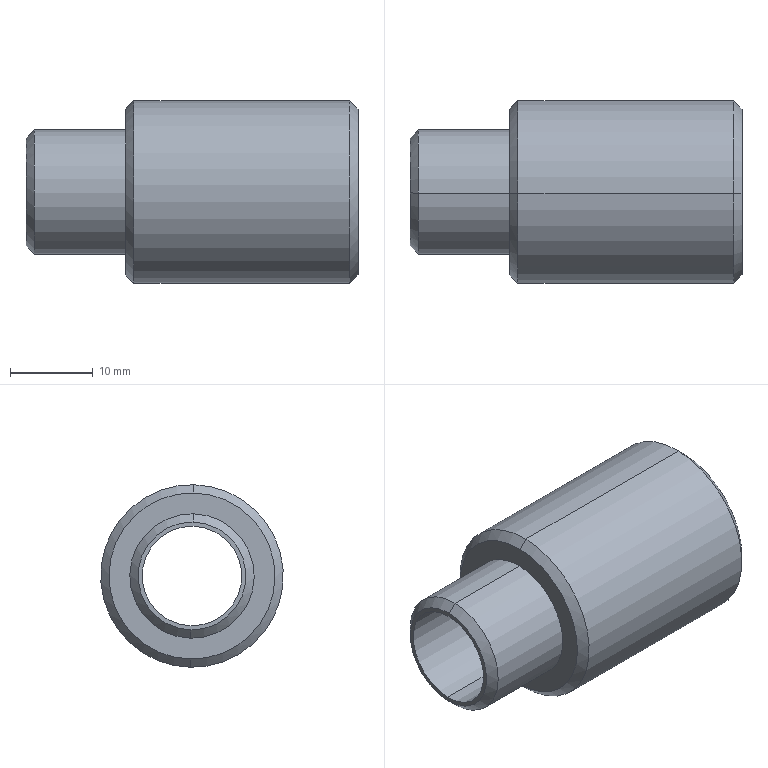Component | SolidWorks | HighVoltageCabinetFrameAssembly-1_FrameFixingSleeve-1 | 1 solid | 18 faces | box 40 x 22 x 22 mm | volume 4758 mm3 | cylinder 8 | cone 6 | plane 4 | commonest cylinder face diameters 18 x2 12 x2 15 x2 22 x2
build123d program:
from build123d import *

# Parameters (mm, degrees)
CHAMFER1_SIZE = 1


with BuildPart() as part:
    # Sketch1 → Revolve1 (revolve)
    with BuildSketch(Plane.XY, mode=Mode.PRIVATE) as revolve1_sk:
        Polygon((0, 11), (28, 11), (28, 7.5), (40, 7.5), (40, 6), (24, 6), (24, 9), (0, 9), align=None)
    revolve(revolve1_sk.sketch.rotate(Axis((0, 0, 0), (1, 0, 0)), 90), axis=Axis((0, 0, 0), (1, 0, 0)))

    # Chamfer1
    chamfer1_edges = [part.edges().sort_by_distance(p)[0] for p in [
        (40, 0, -7.5),
        (28, 0, -11),
        (0, 0, -11),
    ]]
    chamfer(chamfer1_edges, length=CHAMFER1_SIZE)


solid = part.part

# Placed as in the assembly
solid = solid.moved(Location((-1255.437, 161.417, 915.27), (-180, 0, 180)))
STEP:
#1=CARTESIAN_POINT('',(-49.427,6.347,36.428));
#2=VERTEX_POINT('',#1);
#3=CARTESIAN_POINT('',(-49.427,6.363,35.641));
#4=VERTEX_POINT('',#3);
#5=CARTESIAN_POINT('',(-49.427,6.355,36.034));
#6=DIRECTION('',(1.,0.,-0.));
#7=DIRECTION('',(0.,0.01928,-0.9998));
#8=AXIS2_PLACEMENT_3D('',#5,#6,#7);
#9=CIRCLE('',#8,0.3937);
#10=EDGE_CURVE('',#2,#4,#9,.T.);
#11=ORIENTED_EDGE('',*,*,#10,.F.);
#12=CARTESIAN_POINT('',(-49.466,6.347,36.467));
#13=VERTEX_POINT('',#12);
#14=CARTESIAN_POINT('',(-49.427,6.347,36.428));
#15=DIRECTION('',(-0.7071,-0.01364,0.707));
#16=VECTOR('',#15,39.37);
#17=LINE('',#14,#16);
#18=EDGE_CURVE('',#2,#13,#17,.T.);
#19=ORIENTED_EDGE('',*,*,#18,.T.);
#20=CARTESIAN_POINT('',(-49.466,6.363,35.601));
#21=VERTEX_POINT('',#20);
#22=CARTESIAN_POINT('',(-49.466,6.355,36.034));
#23=DIRECTION('',(-1.,-0.,0.));
#24=DIRECTION('',(0.,0.01928,-0.9998));
#25=AXIS2_PLACEMENT_3D('',#22,#23,#24);
#26=CIRCLE('',#25,0.4331);
#27=EDGE_CURVE('',#21,#13,#26,.T.);
#28=ORIENTED_EDGE('',*,*,#27,.F.);
#29=CARTESIAN_POINT('',(-49.427,6.363,35.641));
#30=DIRECTION('',(-0.7071,0.01364,-0.707));
#31=VECTOR('',#30,39.37);
#32=LINE('',#29,#31);
#33=EDGE_CURVE('',#4,#21,#32,.T.);
#34=ORIENTED_EDGE('',*,*,#33,.F.);
#35=EDGE_LOOP('',(#11,#19,#28,#34));
#36=FACE_OUTER_BOUND('',#35,.T.);
#37=CARTESIAN_POINT('',(-49.427,6.355,36.034));
#38=DIRECTION('',(-1.,-0.,0.));
#39=DIRECTION('',(0.,0.01928,-0.9998));
#40=AXIS2_PLACEMENT_3D('',#37,#38,#39);
#41=CONICAL_SURFACE('',#40,0.3937,0.7854);
#42=ADVANCED_FACE('',(#36),#41,.T.);
#43=CARTESIAN_POINT('',(-50.529,6.363,35.641));
#44=VERTEX_POINT('',#43);
#45=CARTESIAN_POINT('',(-50.529,6.347,36.428));
#46=VERTEX_POINT('',#45);
#47=CARTESIAN_POINT('',(-50.529,6.355,36.034));
#48=DIRECTION('',(-1.,-0.,0.));
#49=DIRECTION('',(0.,-0.01928,0.9998));
#50=AXIS2_PLACEMENT_3D('',#47,#48,#49);
#51=CIRCLE('',#50,0.3937);
#52=EDGE_CURVE('',#44,#46,#51,.T.);
#53=ORIENTED_EDGE('',*,*,#52,.F.);
#54=CARTESIAN_POINT('',(-50.49,6.363,35.601));
#55=VERTEX_POINT('',#54);
#56=CARTESIAN_POINT('',(-50.49,6.363,35.601));
#57=DIRECTION('',(0.7071,0.01364,-0.707));
#58=VECTOR('',#57,39.37);
#59=LINE('',#56,#58);
#60=EDGE_CURVE('',#44,#55,#59,.T.);
#61=ORIENTED_EDGE('',*,*,#60,.T.);
#62=CARTESIAN_POINT('',(-50.49,6.347,36.467));
#63=VERTEX_POINT('',#62);
#64=CARTESIAN_POINT('',(-50.49,6.355,36.034));
#65=DIRECTION('',(1.,0.,-0.));
#66=DIRECTION('',(0.,-0.01928,0.9998));
#67=AXIS2_PLACEMENT_3D('',#64,#65,#66);
#68=CIRCLE('',#67,0.4331);
#69=EDGE_CURVE('',#63,#55,#68,.T.);
#70=ORIENTED_EDGE('',*,*,#69,.F.);
#71=CARTESIAN_POINT('',(-50.49,6.347,36.467));
#72=DIRECTION('',(0.7071,-0.01364,0.707));
#73=VECTOR('',#72,39.37);
#74=LINE('',#71,#73);
#75=EDGE_CURVE('',#46,#63,#74,.T.);
#76=ORIENTED_EDGE('',*,*,#75,.F.);
#77=EDGE_LOOP('',(#53,#61,#70,#76));
#78=FACE_OUTER_BOUND('',#77,.T.);
#79=CARTESIAN_POINT('',(-50.49,6.355,36.034));
#80=DIRECTION('',(1.,0.,-0.));
#81=DIRECTION('',(0.,-0.01928,0.9998));
#82=AXIS2_PLACEMENT_3D('',#79,#80,#81);
#83=CONICAL_SURFACE('',#82,0.4331,0.7854);
#84=ADVANCED_FACE('',(#78),#83,.T.);
#85=CARTESIAN_POINT('',(-51.001,6.36,35.778));
#86=VERTEX_POINT('',#85);
#87=CARTESIAN_POINT('',(-51.001,6.35,36.29));
#88=VERTEX_POINT('',#87);
#89=CARTESIAN_POINT('',(-51.001,6.355,36.034));
#90=DIRECTION('',(-1.,-0.,0.));
#91=DIRECTION('',(0.,-0.01928,0.9998));
#92=AXIS2_PLACEMENT_3D('',#89,#90,#91);
#93=CIRCLE('',#92,0.2559);
#94=EDGE_CURVE('',#86,#88,#93,.T.);
#95=ORIENTED_EDGE('',*,*,#94,.F.);
#96=CARTESIAN_POINT('',(-50.962,6.361,35.739));
#97=VERTEX_POINT('',#96);
#98=CARTESIAN_POINT('',(-50.962,6.361,35.739));
#99=DIRECTION('',(0.7071,0.01364,-0.707));
#100=VECTOR('',#99,39.37);
#101=LINE('',#98,#100);
#102=EDGE_CURVE('',#86,#97,#101,.T.);
#103=ORIENTED_EDGE('',*,*,#102,.T.);
#104=CARTESIAN_POINT('',(-50.962,6.349,36.329));
#105=VERTEX_POINT('',#104);
#106=CARTESIAN_POINT('',(-50.962,6.355,36.034));
#107=DIRECTION('',(1.,0.,-0.));
#108=DIRECTION('',(0.,-0.01928,0.9998));
#109=AXIS2_PLACEMENT_3D('',#106,#107,#108);
#110=CIRCLE('',#109,0.2953);
#111=EDGE_CURVE('',#105,#97,#110,.T.);
#112=ORIENTED_EDGE('',*,*,#111,.F.);
#113=CARTESIAN_POINT('',(-50.962,6.349,36.329));
#114=DIRECTION('',(0.7071,-0.01364,0.707));
#115=VECTOR('',#114,39.37);
#116=LINE('',#113,#115);
#117=EDGE_CURVE('',#88,#105,#116,.T.);
#118=ORIENTED_EDGE('',*,*,#117,.F.);
#119=EDGE_LOOP('',(#95,#103,#112,#118));
#120=FACE_OUTER_BOUND('',#119,.T.);
#121=CARTESIAN_POINT('',(-50.962,6.355,36.034));
#122=DIRECTION('',(1.,0.,-0.));
#123=DIRECTION('',(0.,-0.01928,0.9998));
#124=AXIS2_PLACEMENT_3D('',#121,#122,#123);
#125=CONICAL_SURFACE('',#124,0.2953,0.7854);
#126=ADVANCED_FACE('',(#120),#125,.T.);
#127=CARTESIAN_POINT('',(-50.372,6.362,35.68));
#128=VERTEX_POINT('',#127);
#129=CARTESIAN_POINT('',(-50.372,6.348,36.389));
#130=VERTEX_POINT('',#129);
#131=CARTESIAN_POINT('',(-50.372,6.355,36.034));
#132=DIRECTION('',(1.,0.,-0.));
#133=DIRECTION('',(0.,-0.01928,0.9998));
#134=AXIS2_PLACEMENT_3D('',#131,#132,#133);
#135=CIRCLE('',#134,0.3543);
#136=EDGE_CURVE('',#128,#130,#135,.T.);
#137=ORIENTED_EDGE('',*,*,#136,.F.);
#138=CARTESIAN_POINT('',(-49.427,6.362,35.68));
#139=VERTEX_POINT('',#138);
#140=CARTESIAN_POINT('',(-49.427,6.362,35.68));
#141=DIRECTION('',(1.,0.,-0.));
#142=VECTOR('',#141,39.37);
#143=LINE('',#140,#142);
#144=EDGE_CURVE('',#128,#139,#143,.T.);
#145=ORIENTED_EDGE('',*,*,#144,.T.);
#146=CARTESIAN_POINT('',(-49.427,6.348,36.389));
#147=VERTEX_POINT('',#146);
#148=CARTESIAN_POINT('',(-49.427,6.355,36.034));
#149=DIRECTION('',(1.,0.,-0.));
#150=DIRECTION('',(0.,-0.01928,0.9998));
#151=AXIS2_PLACEMENT_3D('',#148,#149,#150);
#152=CIRCLE('',#151,0.3543);
#153=EDGE_CURVE('',#139,#147,#152,.T.);
#154=ORIENTED_EDGE('',*,*,#153,.T.);
#155=CARTESIAN_POINT('',(-49.427,6.348,36.389));
#156=DIRECTION('',(1.,0.,-0.));
#157=VECTOR('',#156,39.37);
#158=LINE('',#155,#157);
#159=EDGE_CURVE('',#130,#147,#158,.T.);
#160=ORIENTED_EDGE('',*,*,#159,.F.);
#161=EDGE_LOOP('',(#137,#145,#154,#160));
#162=FACE_OUTER_BOUND('',#161,.T.);
#163=CARTESIAN_POINT('',(-49.427,6.355,36.034));
#164=DIRECTION('',(1.,0.,-0.));
#165=DIRECTION('',(0.,-0.01928,0.9998));
#166=AXIS2_PLACEMENT_3D('',#163,#164,#165);
#167=CYLINDRICAL_SURFACE('',#166,0.3543);
#168=ADVANCED_FACE('',(#162),#167,.F.);
#169=CARTESIAN_POINT('',(-51.001,6.36,35.798));
#170=VERTEX_POINT('',#169);
#171=CARTESIAN_POINT('',(-51.001,6.35,36.27));
#172=VERTEX_POINT('',#171);
#173=CARTESIAN_POINT('',(-51.001,6.355,36.034));
#174=DIRECTION('',(1.,0.,-0.));
#175=DIRECTION('',(0.,-0.01928,0.9998));
#176=AXIS2_PLACEMENT_3D('',#173,#174,#175);
#177=CIRCLE('',#176,0.2362);
#178=EDGE_CURVE('',#170,#172,#177,.T.);
#179=ORIENTED_EDGE('',*,*,#178,.F.);
#180=CARTESIAN_POINT('',(-50.372,6.36,35.798));
#181=VERTEX_POINT('',#180);
#182=CARTESIAN_POINT('',(-49.427,6.36,35.798));
#183=DIRECTION('',(1.,0.,-0.));
#184=VECTOR('',#183,39.37);
#185=LINE('',#182,#184);
#186=EDGE_CURVE('',#170,#181,#185,.T.);
#187=ORIENTED_EDGE('',*,*,#186,.T.);
#188=CARTESIAN_POINT('',(-50.372,6.35,36.27));
#189=VERTEX_POINT('',#188);
#190=CARTESIAN_POINT('',(-50.372,6.355,36.034));
#191=DIRECTION('',(1.,0.,-0.));
#192=DIRECTION('',(0.,-0.01928,0.9998));
#193=AXIS2_PLACEMENT_3D('',#190,#191,#192);
#194=CIRCLE('',#193,0.2362);
#195=EDGE_CURVE('',#181,#189,#194,.T.);
#196=ORIENTED_EDGE('',*,*,#195,.T.);
#197=CARTESIAN_POINT('',(-49.427,6.35,36.27));
#198=DIRECTION('',(1.,0.,-0.));
#199=VECTOR('',#198,39.37);
#200=LINE('',#197,#199);
#201=EDGE_CURVE('',#172,#189,#200,.T.);
#202=ORIENTED_EDGE('',*,*,#201,.F.);
#203=EDGE_LOOP('',(#179,#187,#196,#202));
#204=FACE_OUTER_BOUND('',#203,.T.);
#205=CARTESIAN_POINT('',(-49.427,6.355,36.034));
#206=DIRECTION('',(1.,0.,-0.));
#207=DIRECTION('',(0.,-0.01928,0.9998));
#208=AXIS2_PLACEMENT_3D('',#205,#206,#207);
#209=CYLINDRICAL_SURFACE('',#208,0.2362);
#210=ADVANCED_FACE('',(#204),#209,.F.);
#211=ORIENTED_EDGE('',*,*,#111,.T.);
#212=CARTESIAN_POINT('',(-50.529,6.361,35.739));
#213=VERTEX_POINT('',#212);
#214=CARTESIAN_POINT('',(-49.427,6.361,35.739));
#215=DIRECTION('',(1.,0.,-0.));
#216=VECTOR('',#215,39.37);
#217=LINE('',#214,#216);
#218=EDGE_CURVE('',#97,#213,#217,.T.);
#219=ORIENTED_EDGE('',*,*,#218,.T.);
#220=CARTESIAN_POINT('',(-50.529,6.349,36.329));
#221=VERTEX_POINT('',#220);
#222=CARTESIAN_POINT('',(-50.529,6.355,36.034));
#223=DIRECTION('',(1.,0.,-0.));
#224=DIRECTION('',(0.,-0.01928,0.9998));
#225=AXIS2_PLACEMENT_3D('',#222,#223,#224);
#226=CIRCLE('',#225,0.2953);
#227=EDGE_CURVE('',#221,#213,#226,.T.);
#228=ORIENTED_EDGE('',*,*,#227,.F.);
#229=CARTESIAN_POINT('',(-49.427,6.349,36.329));
#230=DIRECTION('',(1.,0.,-0.));
#231=VECTOR('',#230,39.37);
#232=LINE('',#229,#231);
#233=EDGE_CURVE('',#105,#221,#232,.T.);
#234=ORIENTED_EDGE('',*,*,#233,.F.);
#235=EDGE_LOOP('',(#211,#219,#228,#234));
#236=FACE_OUTER_BOUND('',#235,.T.);
#237=CARTESIAN_POINT('',(-49.427,6.355,36.034));
#238=DIRECTION('',(1.,0.,-0.));
#239=DIRECTION('',(0.,-0.01928,0.9998));
#240=AXIS2_PLACEMENT_3D('',#237,#238,#239);
#241=CYLINDRICAL_SURFACE('',#240,0.2953);
#242=ADVANCED_FACE('',(#236),#241,.T.);
#243=ORIENTED_EDGE('',*,*,#69,.T.);
#244=CARTESIAN_POINT('',(-49.427,6.363,35.601));
#245=DIRECTION('',(1.,0.,-0.));
#246=VECTOR('',#245,39.37);
#247=LINE('',#244,#246);
#248=EDGE_CURVE('',#55,#21,#247,.T.);
#249=ORIENTED_EDGE('',*,*,#248,.T.);
#250=ORIENTED_EDGE('',*,*,#27,.T.);
#251=CARTESIAN_POINT('',(-49.427,6.347,36.467));
#252=DIRECTION('',(1.,0.,-0.));
#253=VECTOR('',#252,39.37);
#254=LINE('',#251,#253);
#255=EDGE_CURVE('',#63,#13,#254,.T.);
#256=ORIENTED_EDGE('',*,*,#255,.F.);
#257=EDGE_LOOP('',(#243,#249,#250,#256));
#258=FACE_OUTER_BOUND('',#257,.T.);
#259=CARTESIAN_POINT('',(-49.427,6.355,36.034));
#260=DIRECTION('',(1.,0.,-0.));
#261=DIRECTION('',(0.,-0.01928,0.9998));
#262=AXIS2_PLACEMENT_3D('',#259,#260,#261);
#263=CYLINDRICAL_SURFACE('',#262,0.4331);
#264=ADVANCED_FACE('',(#258),#263,.T.);
#265=CARTESIAN_POINT('',(-49.427,6.355,36.034));
#266=DIRECTION('',(1.,0.,-0.));
#267=DIRECTION('',(0.,0.01928,-0.9998));
#268=AXIS2_PLACEMENT_3D('',#265,#266,#267);
#269=CIRCLE('',#268,0.3937);
#270=EDGE_CURVE('',#4,#2,#269,.T.);
#271=ORIENTED_EDGE('',*,*,#270,.T.);
#272=ORIENTED_EDGE('',*,*,#10,.T.);
#273=EDGE_LOOP('',(#271,#272));
#274=FACE_OUTER_BOUND('',#273,.T.);
#275=CARTESIAN_POINT('',(-49.427,6.355,36.034));
#276=DIRECTION('',(1.,0.,-0.));
#277=DIRECTION('',(0.,-0.01928,0.9998));
#278=AXIS2_PLACEMENT_3D('',#275,#276,#277);
#279=CIRCLE('',#278,0.3543);
#280=EDGE_CURVE('',#147,#139,#279,.T.);
#281=ORIENTED_EDGE('',*,*,#280,.F.);
#282=ORIENTED_EDGE('',*,*,#153,.F.);
#283=EDGE_LOOP('',(#281,#282));
#284=FACE_BOUND('',#283,.T.);
#285=CARTESIAN_POINT('',(-49.427,6.001,36.027));
#286=DIRECTION('',(-1.,-0.,-0.));
#287=DIRECTION('',(0.,0.01928,-0.9998));
#288=AXIS2_PLACEMENT_3D('',#285,#286,#287);
#289=PLANE('',#288);
#290=ADVANCED_FACE('',(#274,#284),#289,.F.);
#291=ORIENTED_EDGE('',*,*,#248,.F.);
#292=CARTESIAN_POINT('',(-50.49,6.355,36.034));
#293=DIRECTION('',(1.,0.,-0.));
#294=DIRECTION('',(0.,-0.01928,0.9998));
#295=AXIS2_PLACEMENT_3D('',#292,#293,#294);
#296=CIRCLE('',#295,0.4331);
#297=EDGE_CURVE('',#55,#63,#296,.T.);
#298=ORIENTED_EDGE('',*,*,#297,.T.);
#299=ORIENTED_EDGE('',*,*,#255,.T.);
#300=CARTESIAN_POINT('',(-49.466,6.355,36.034));
#301=DIRECTION('',(-1.,-0.,0.));
#302=DIRECTION('',(0.,0.01928,-0.9998));
#303=AXIS2_PLACEMENT_3D('',#300,#301,#302);
#304=CIRCLE('',#303,0.4331);
#305=EDGE_CURVE('',#13,#21,#304,.T.);
#306=ORIENTED_EDGE('',*,*,#305,.T.);
#307=EDGE_LOOP('',(#291,#298,#299,#306));
#308=FACE_OUTER_BOUND('',#307,.T.);
#309=CARTESIAN_POINT('',(-49.427,6.355,36.034));
#310=DIRECTION('',(1.,0.,-0.));
#311=DIRECTION('',(0.,-0.01928,0.9998));
#312=AXIS2_PLACEMENT_3D('',#309,#310,#311);
#313=CYLINDRICAL_SURFACE('',#312,0.4331);
#314=ADVANCED_FACE('',(#308),#313,.T.);
#315=CARTESIAN_POINT('',(-50.529,6.355,36.034));
#316=DIRECTION('',(-1.,-0.,0.));
#317=DIRECTION('',(0.,-0.01928,0.9998));
#318=AXIS2_PLACEMENT_3D('',#315,#316,#317);
#319=CIRCLE('',#318,0.3937);
#320=EDGE_CURVE('',#46,#44,#319,.T.);
#321=ORIENTED_EDGE('',*,*,#320,.T.);
#322=ORIENTED_EDGE('',*,*,#52,.T.);
#323=EDGE_LOOP('',(#321,#322));
#324=FACE_OUTER_BOUND('',#323,.T.);
#325=ORIENTED_EDGE('',*,*,#227,.T.);
#326=CARTESIAN_POINT('',(-50.529,6.355,36.034));
#327=DIRECTION('',(1.,0.,-0.));
#328=DIRECTION('',(0.,-0.01928,0.9998));
#329=AXIS2_PLACEMENT_3D('',#326,#327,#328);
#330=CIRCLE('',#329,0.2953);
#331=EDGE_CURVE('',#213,#221,#330,.T.);
#332=ORIENTED_EDGE('',*,*,#331,.T.);
#333=EDGE_LOOP('',(#325,#332));
#334=FACE_BOUND('',#333,.T.);
#335=CARTESIAN_POINT('',(-50.529,5.922,36.026));
#336=DIRECTION('',(1.,0.,0.));
#337=DIRECTION('',(-0.,-0.01928,0.9998));
#338=AXIS2_PLACEMENT_3D('',#335,#336,#337);
#339=PLANE('',#338);
#340=ADVANCED_FACE('',(#324,#334),#339,.F.);
#341=ORIENTED_EDGE('',*,*,#218,.F.);
#342=CARTESIAN_POINT('',(-50.962,6.355,36.034));
#343=DIRECTION('',(1.,0.,-0.));
#344=DIRECTION('',(0.,-0.01928,0.9998));
#345=AXIS2_PLACEMENT_3D('',#342,#343,#344);
#346=CIRCLE('',#345,0.2953);
#347=EDGE_CURVE('',#97,#105,#346,.T.);
#348=ORIENTED_EDGE('',*,*,#347,.T.);
#349=ORIENTED_EDGE('',*,*,#233,.T.);
#350=ORIENTED_EDGE('',*,*,#331,.F.);
#351=EDGE_LOOP('',(#341,#348,#349,#350));
#352=FACE_OUTER_BOUND('',#351,.T.);
#353=CARTESIAN_POINT('',(-49.427,6.355,36.034));
#354=DIRECTION('',(1.,0.,-0.));
#355=DIRECTION('',(0.,-0.01928,0.9998));
#356=AXIS2_PLACEMENT_3D('',#353,#354,#355);
#357=CYLINDRICAL_SURFACE('',#356,0.2953);
#358=ADVANCED_FACE('',(#352),#357,.T.);
#359=CARTESIAN_POINT('',(-51.001,6.355,36.034));
#360=DIRECTION('',(-1.,-0.,0.));
#361=DIRECTION('',(0.,-0.01928,0.9998));
#362=AXIS2_PLACEMENT_3D('',#359,#360,#361);
#363=CIRCLE('',#362,0.2559);
#364=EDGE_CURVE('',#88,#86,#363,.T.);
#365=ORIENTED_EDGE('',*,*,#364,.T.);
#366=ORIENTED_EDGE('',*,*,#94,.T.);
#367=EDGE_LOOP('',(#365,#366));
#368=FACE_OUTER_BOUND('',#367,.T.);
#369=CARTESIAN_POINT('',(-51.001,6.355,36.034));
#370=DIRECTION('',(1.,0.,-0.));
#371=DIRECTION('',(0.,-0.01928,0.9998));
#372=AXIS2_PLACEMENT_3D('',#369,#370,#371);
#373=CIRCLE('',#372,0.2362);
#374=EDGE_CURVE('',#172,#170,#373,.T.);
#375=ORIENTED_EDGE('',*,*,#374,.T.);
#376=ORIENTED_EDGE('',*,*,#178,.T.);
#377=EDGE_LOOP('',(#375,#376));
#378=FACE_BOUND('',#377,.T.);
#379=CARTESIAN_POINT('',(-51.001,6.06,36.029));
#380=DIRECTION('',(1.,0.,0.));
#381=DIRECTION('',(-0.,-0.01928,0.9998));
#382=AXIS2_PLACEMENT_3D('',#379,#380,#381);
#383=PLANE('',#382);
#384=ADVANCED_FACE('',(#368,#378),#383,.F.);
#385=ORIENTED_EDGE('',*,*,#186,.F.);
#386=ORIENTED_EDGE('',*,*,#374,.F.);
#387=ORIENTED_EDGE('',*,*,#201,.T.);
#388=CARTESIAN_POINT('',(-50.372,6.355,36.034));
#389=DIRECTION('',(1.,0.,-0.));
#390=DIRECTION('',(0.,-0.01928,0.9998));
#391=AXIS2_PLACEMENT_3D('',#388,#389,#390);
#392=CIRCLE('',#391,0.2362);
#393=EDGE_CURVE('',#189,#181,#392,.T.);
#394=ORIENTED_EDGE('',*,*,#393,.T.);
#395=EDGE_LOOP('',(#385,#386,#387,#394));
#396=FACE_OUTER_BOUND('',#395,.T.);
#397=CARTESIAN_POINT('',(-49.427,6.355,36.034));
#398=DIRECTION('',(1.,0.,-0.));
#399=DIRECTION('',(0.,-0.01928,0.9998));
#400=AXIS2_PLACEMENT_3D('',#397,#398,#399);
#401=CYLINDRICAL_SURFACE('',#400,0.2362);
#402=ADVANCED_FACE('',(#396),#401,.F.);
#403=ORIENTED_EDGE('',*,*,#393,.F.);
#404=ORIENTED_EDGE('',*,*,#195,.F.);
#405=EDGE_LOOP('',(#403,#404));
#406=FACE_BOUND('',#405,.T.);
#407=CARTESIAN_POINT('',(-50.372,6.355,36.034));
#408=DIRECTION('',(1.,0.,-0.));
#409=DIRECTION('',(0.,-0.01928,0.9998));
#410=AXIS2_PLACEMENT_3D('',#407,#408,#409);
#411=CIRCLE('',#410,0.3543);
#412=EDGE_CURVE('',#130,#128,#411,.T.);
#413=ORIENTED_EDGE('',*,*,#412,.T.);
#414=ORIENTED_EDGE('',*,*,#136,.T.);
#415=EDGE_LOOP('',(#413,#414));
#416=FACE_OUTER_BOUND('',#415,.T.);
#417=CARTESIAN_POINT('',(-50.372,6.119,36.03));
#418=DIRECTION('',(-1.,-0.,-0.));
#419=DIRECTION('',(0.,0.01928,-0.9998));
#420=AXIS2_PLACEMENT_3D('',#417,#418,#419);
#421=PLANE('',#420);
#422=ADVANCED_FACE('',(#406,#416),#421,.F.);
#423=ORIENTED_EDGE('',*,*,#144,.F.);
#424=ORIENTED_EDGE('',*,*,#412,.F.);
#425=ORIENTED_EDGE('',*,*,#159,.T.);
#426=ORIENTED_EDGE('',*,*,#280,.T.);
#427=EDGE_LOOP('',(#423,#424,#425,#426));
#428=FACE_OUTER_BOUND('',#427,.T.);
#429=CARTESIAN_POINT('',(-49.427,6.355,36.034));
#430=DIRECTION('',(1.,0.,-0.));
#431=DIRECTION('',(0.,-0.01928,0.9998));
#432=AXIS2_PLACEMENT_3D('',#429,#430,#431);
#433=CYLINDRICAL_SURFACE('',#432,0.3543);
#434=ADVANCED_FACE('',(#428),#433,.F.);
#435=ORIENTED_EDGE('',*,*,#102,.F.);
#436=ORIENTED_EDGE('',*,*,#364,.F.);
#437=ORIENTED_EDGE('',*,*,#117,.T.);
#438=ORIENTED_EDGE('',*,*,#347,.F.);
#439=EDGE_LOOP('',(#435,#436,#437,#438));
#440=FACE_OUTER_BOUND('',#439,.T.);
#441=CARTESIAN_POINT('',(-50.962,6.355,36.034));
#442=DIRECTION('',(1.,0.,-0.));
#443=DIRECTION('',(0.,-0.01928,0.9998));
#444=AXIS2_PLACEMENT_3D('',#441,#442,#443);
#445=CONICAL_SURFACE('',#444,0.2953,0.7854);
#446=ADVANCED_FACE('',(#440),#445,.T.);
#447=ORIENTED_EDGE('',*,*,#60,.F.);
#448=ORIENTED_EDGE('',*,*,#320,.F.);
#449=ORIENTED_EDGE('',*,*,#75,.T.);
#450=ORIENTED_EDGE('',*,*,#297,.F.);
#451=EDGE_LOOP('',(#447,#448,#449,#450));
#452=FACE_OUTER_BOUND('',#451,.T.);
#453=CARTESIAN_POINT('',(-50.49,6.355,36.034));
#454=DIRECTION('',(1.,0.,-0.));
#455=DIRECTION('',(0.,-0.01928,0.9998));
#456=AXIS2_PLACEMENT_3D('',#453,#454,#455);
#457=CONICAL_SURFACE('',#456,0.4331,0.7854);
#458=ADVANCED_FACE('',(#452),#457,.T.);
#459=ORIENTED_EDGE('',*,*,#18,.F.);
#460=ORIENTED_EDGE('',*,*,#270,.F.);
#461=ORIENTED_EDGE('',*,*,#33,.T.);
#462=ORIENTED_EDGE('',*,*,#305,.F.);
#463=EDGE_LOOP('',(#459,#460,#461,#462));
#464=FACE_OUTER_BOUND('',#463,.T.);
#465=CARTESIAN_POINT('',(-49.427,6.355,36.034));
#466=DIRECTION('',(-1.,-0.,0.));
#467=DIRECTION('',(0.,0.01928,-0.9998));
#468=AXIS2_PLACEMENT_3D('',#465,#466,#467);
#469=CONICAL_SURFACE('',#468,0.3937,0.7854);
#470=ADVANCED_FACE('',(#464),#469,.T.);
#471=CLOSED_SHELL('',(#42,#84,#126,#168,#210,#242,#264,#290,#314,#340,#358,#384,#402,#422,#434,#446,#458,#470));
#472=MANIFOLD_SOLID_BREP('',#471);
#473=CARTESIAN_POINT('',(0.,0.,0.));
#474=DIRECTION('',(0.,0.,1.));
#475=DIRECTION('',(1.,0.,0.));
#476=AXIS2_PLACEMENT_3D('',#473,#474,#475);
#477=(LENGTH_UNIT()NAMED_UNIT(*)SI_UNIT($,.METRE.));
#478=LENGTH_MEASURE_WITH_UNIT(LENGTH_MEASURE(0.0254),#477);
#479=DIMENSIONAL_EXPONENTS(1.,0.,0.,0.,0.,0.,0.);
#480=(CONVERSION_BASED_UNIT('',#478)LENGTH_UNIT()NAMED_UNIT(#479));
#481=UNCERTAINTY_MEASURE_WITH_UNIT(LENGTH_MEASURE(0.00001),#480,'','');
#482=(NAMED_UNIT(*)PLANE_ANGLE_UNIT()SI_UNIT($,.RADIAN.));
#483=(NAMED_UNIT(*)SI_UNIT($,.STERADIAN.)SOLID_ANGLE_UNIT());
#484=(GEOMETRIC_REPRESENTATION_CONTEXT(3)GLOBAL_UNCERTAINTY_ASSIGNED_CONTEXT((#481))GLOBAL_UNIT_ASSIGNED_CONTEXT((#480,#482,#483))REPRESENTATION_CONTEXT('',''));
#485=ADVANCED_BREP_SHAPE_REPRESENTATION('',(#472,#476),#484);
#486=COLOUR_RGB('',0.7922,0.8196,0.9333);
#487=FILL_AREA_STYLE_COLOUR('',#486);
#488=FILL_AREA_STYLE('',(#487));
#489=SURFACE_STYLE_FILL_AREA(#488);
#490=SURFACE_SIDE_STYLE('',(#489));
#491=SURFACE_STYLE_USAGE(.BOTH.,#490);
#492=PRESENTATION_STYLE_ASSIGNMENT((#491));
#493=STYLED_ITEM('',(#492),#472);
#494=(LENGTH_UNIT()NAMED_UNIT(*)SI_UNIT($,.METRE.));
#495=LENGTH_MEASURE_WITH_UNIT(LENGTH_MEASURE(0.0254),#494);
#496=DIMENSIONAL_EXPONENTS(1.,0.,0.,0.,0.,0.,0.);
#497=(CONVERSION_BASED_UNIT('',#495)LENGTH_UNIT()NAMED_UNIT(#496));
#498=UNCERTAINTY_MEASURE_WITH_UNIT(LENGTH_MEASURE(0.00001),#497,'','');
#499=(NAMED_UNIT(*)PLANE_ANGLE_UNIT()SI_UNIT($,.RADIAN.));
#500=(NAMED_UNIT(*)SI_UNIT($,.STERADIAN.)SOLID_ANGLE_UNIT());
#501=(GEOMETRIC_REPRESENTATION_CONTEXT(3)GLOBAL_UNCERTAINTY_ASSIGNED_CONTEXT((#498))GLOBAL_UNIT_ASSIGNED_CONTEXT((#497,#499,#500))REPRESENTATION_CONTEXT('',''));
#502=MECHANICAL_DESIGN_GEOMETRIC_PRESENTATION_REPRESENTATION('',(#493),#501);
#503=PRESENTATION_LAYER_ASSIGNMENT('','',(#493));